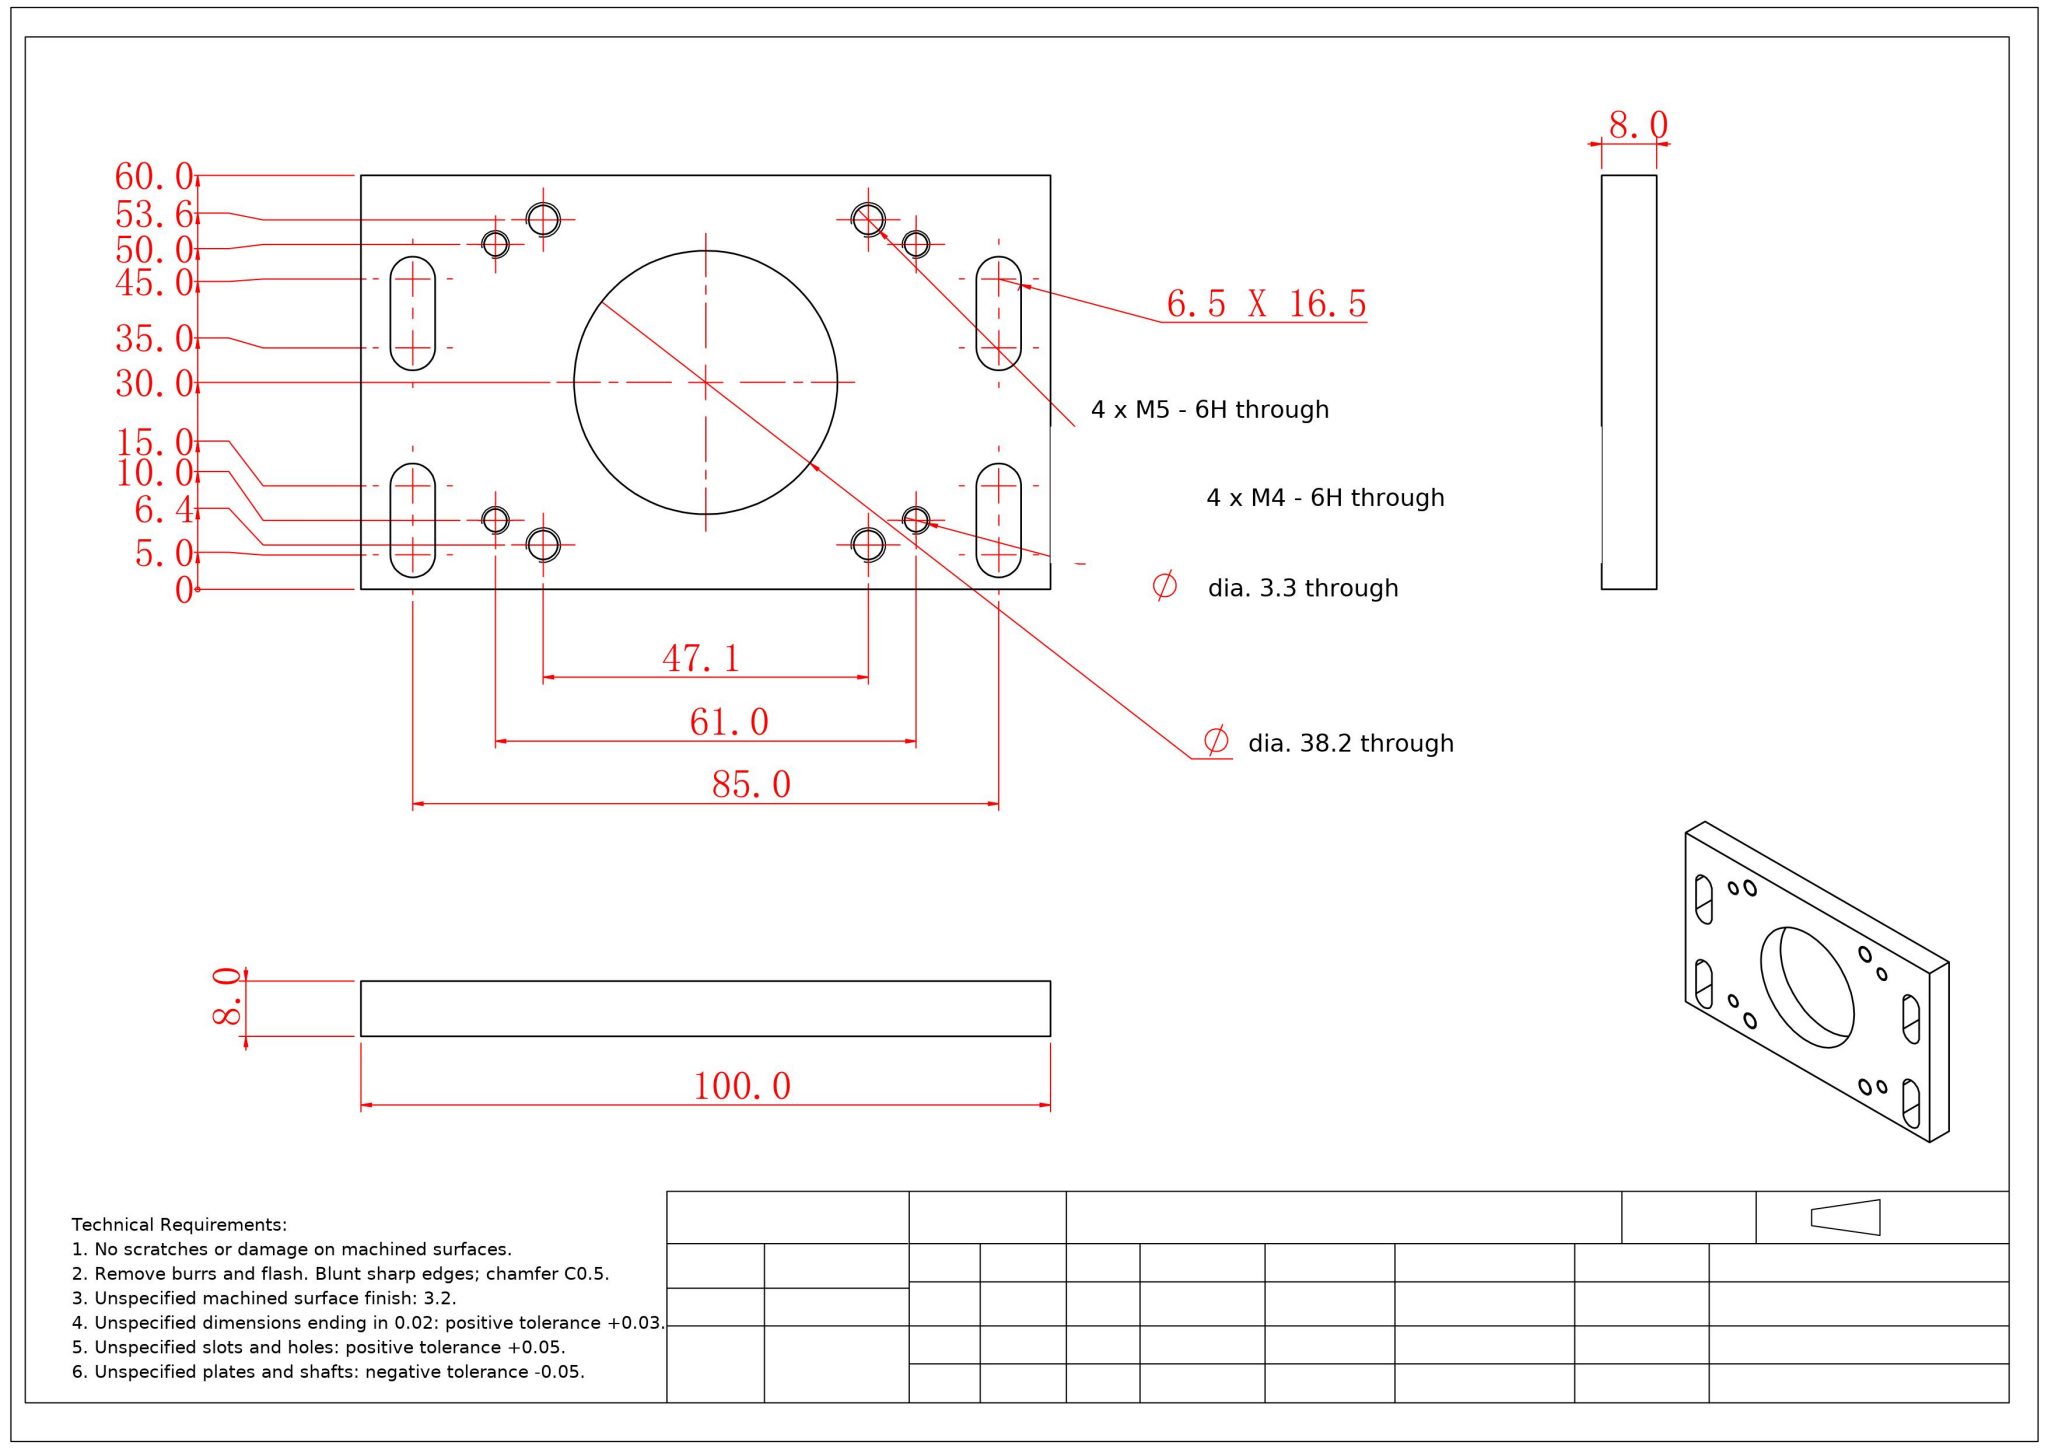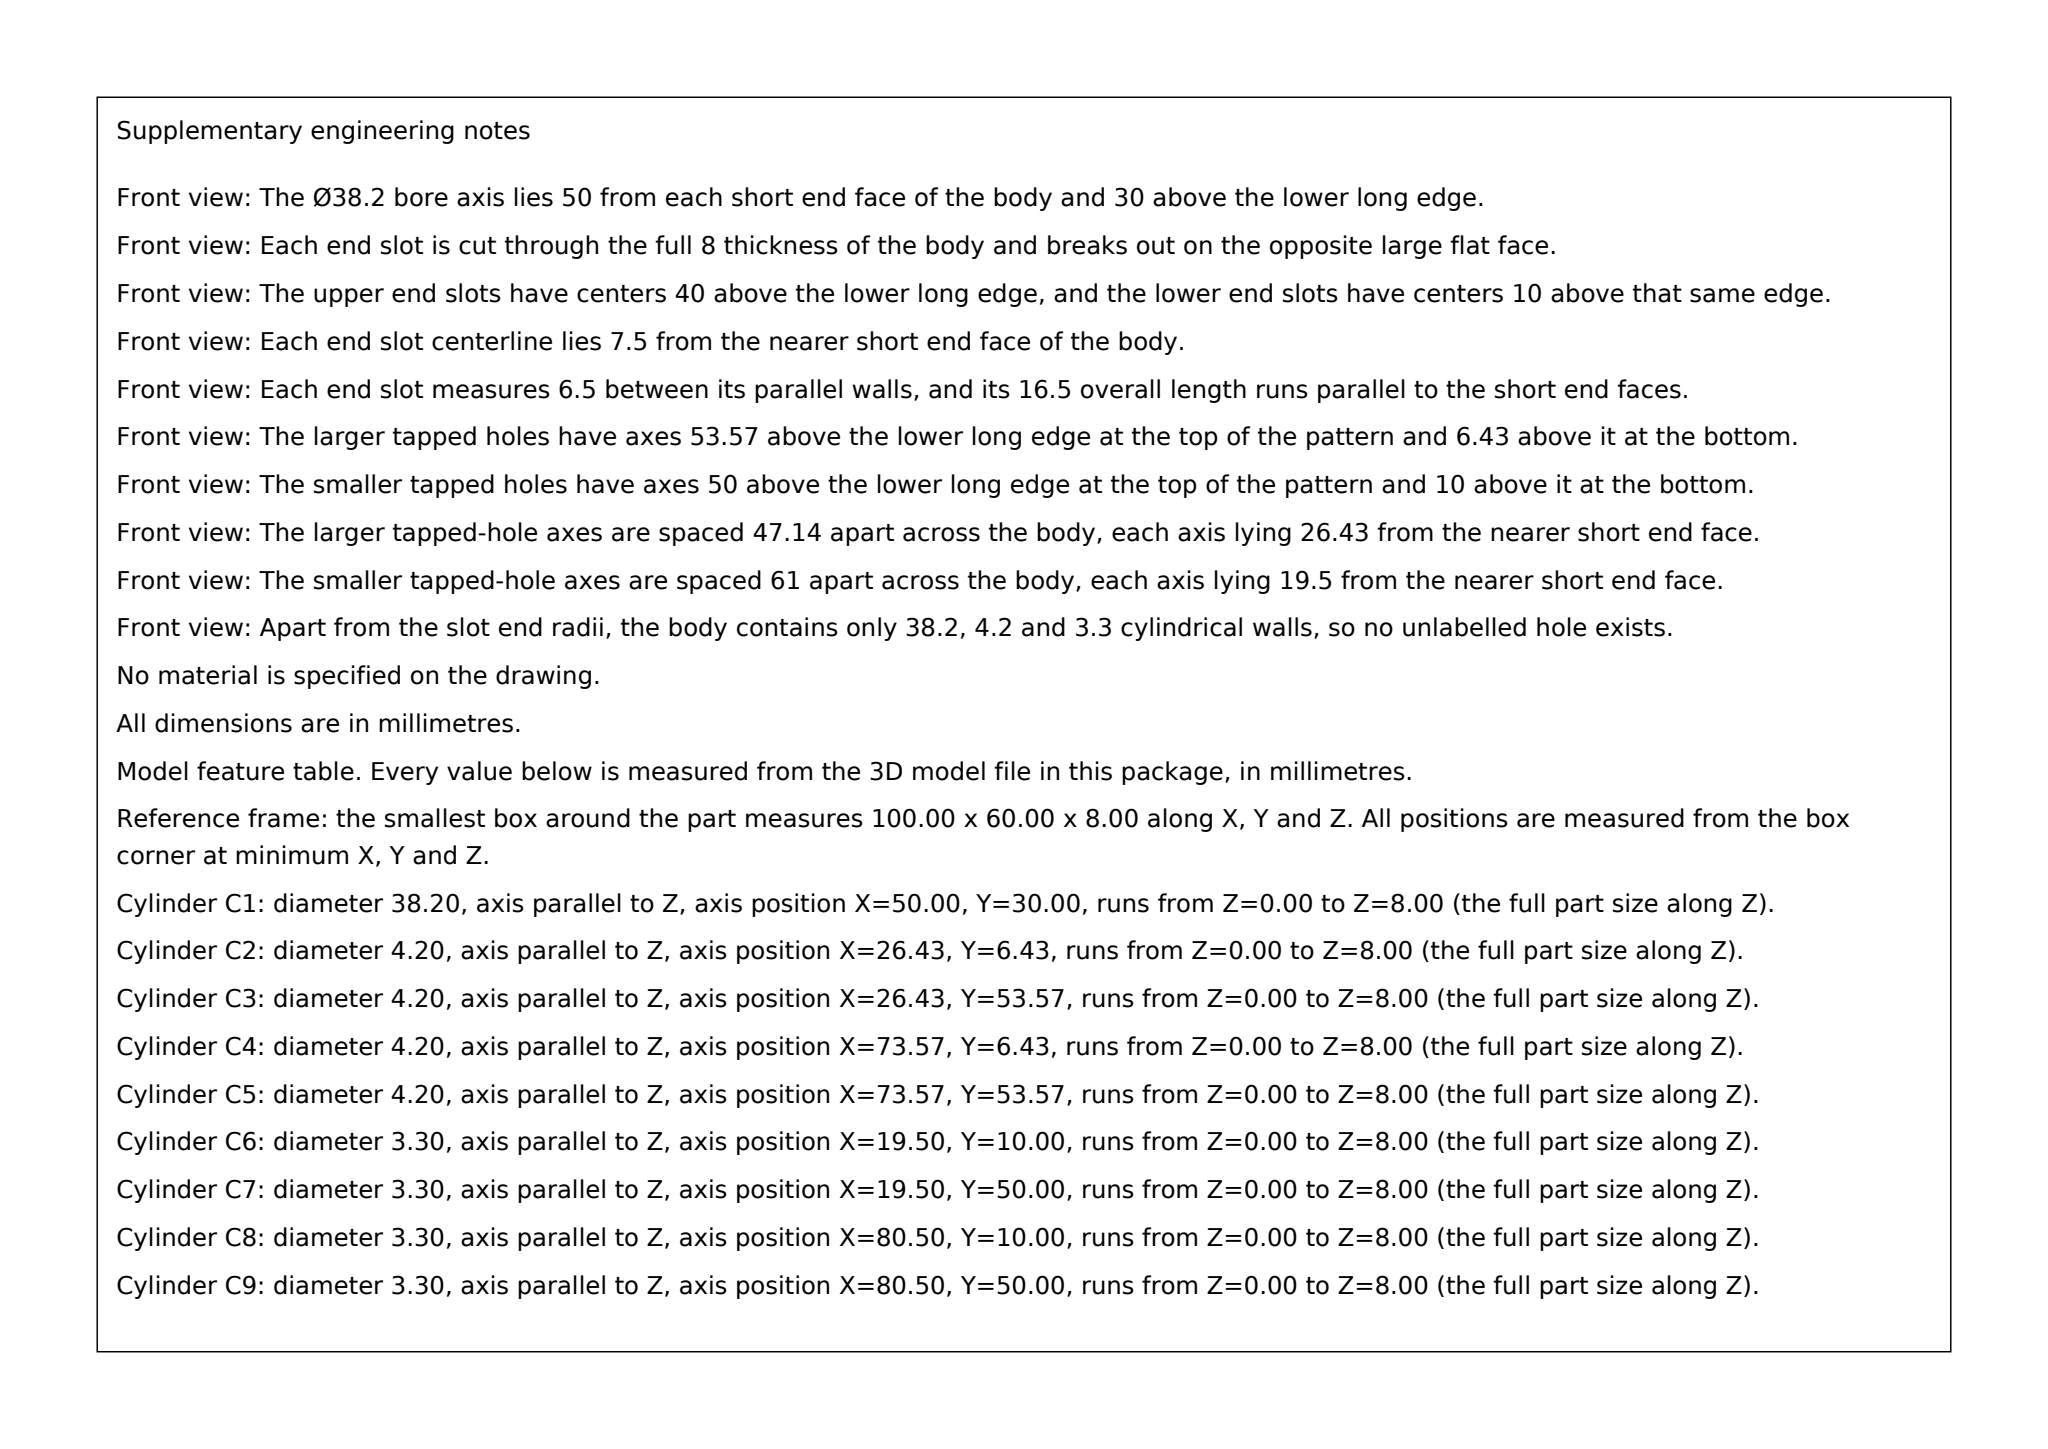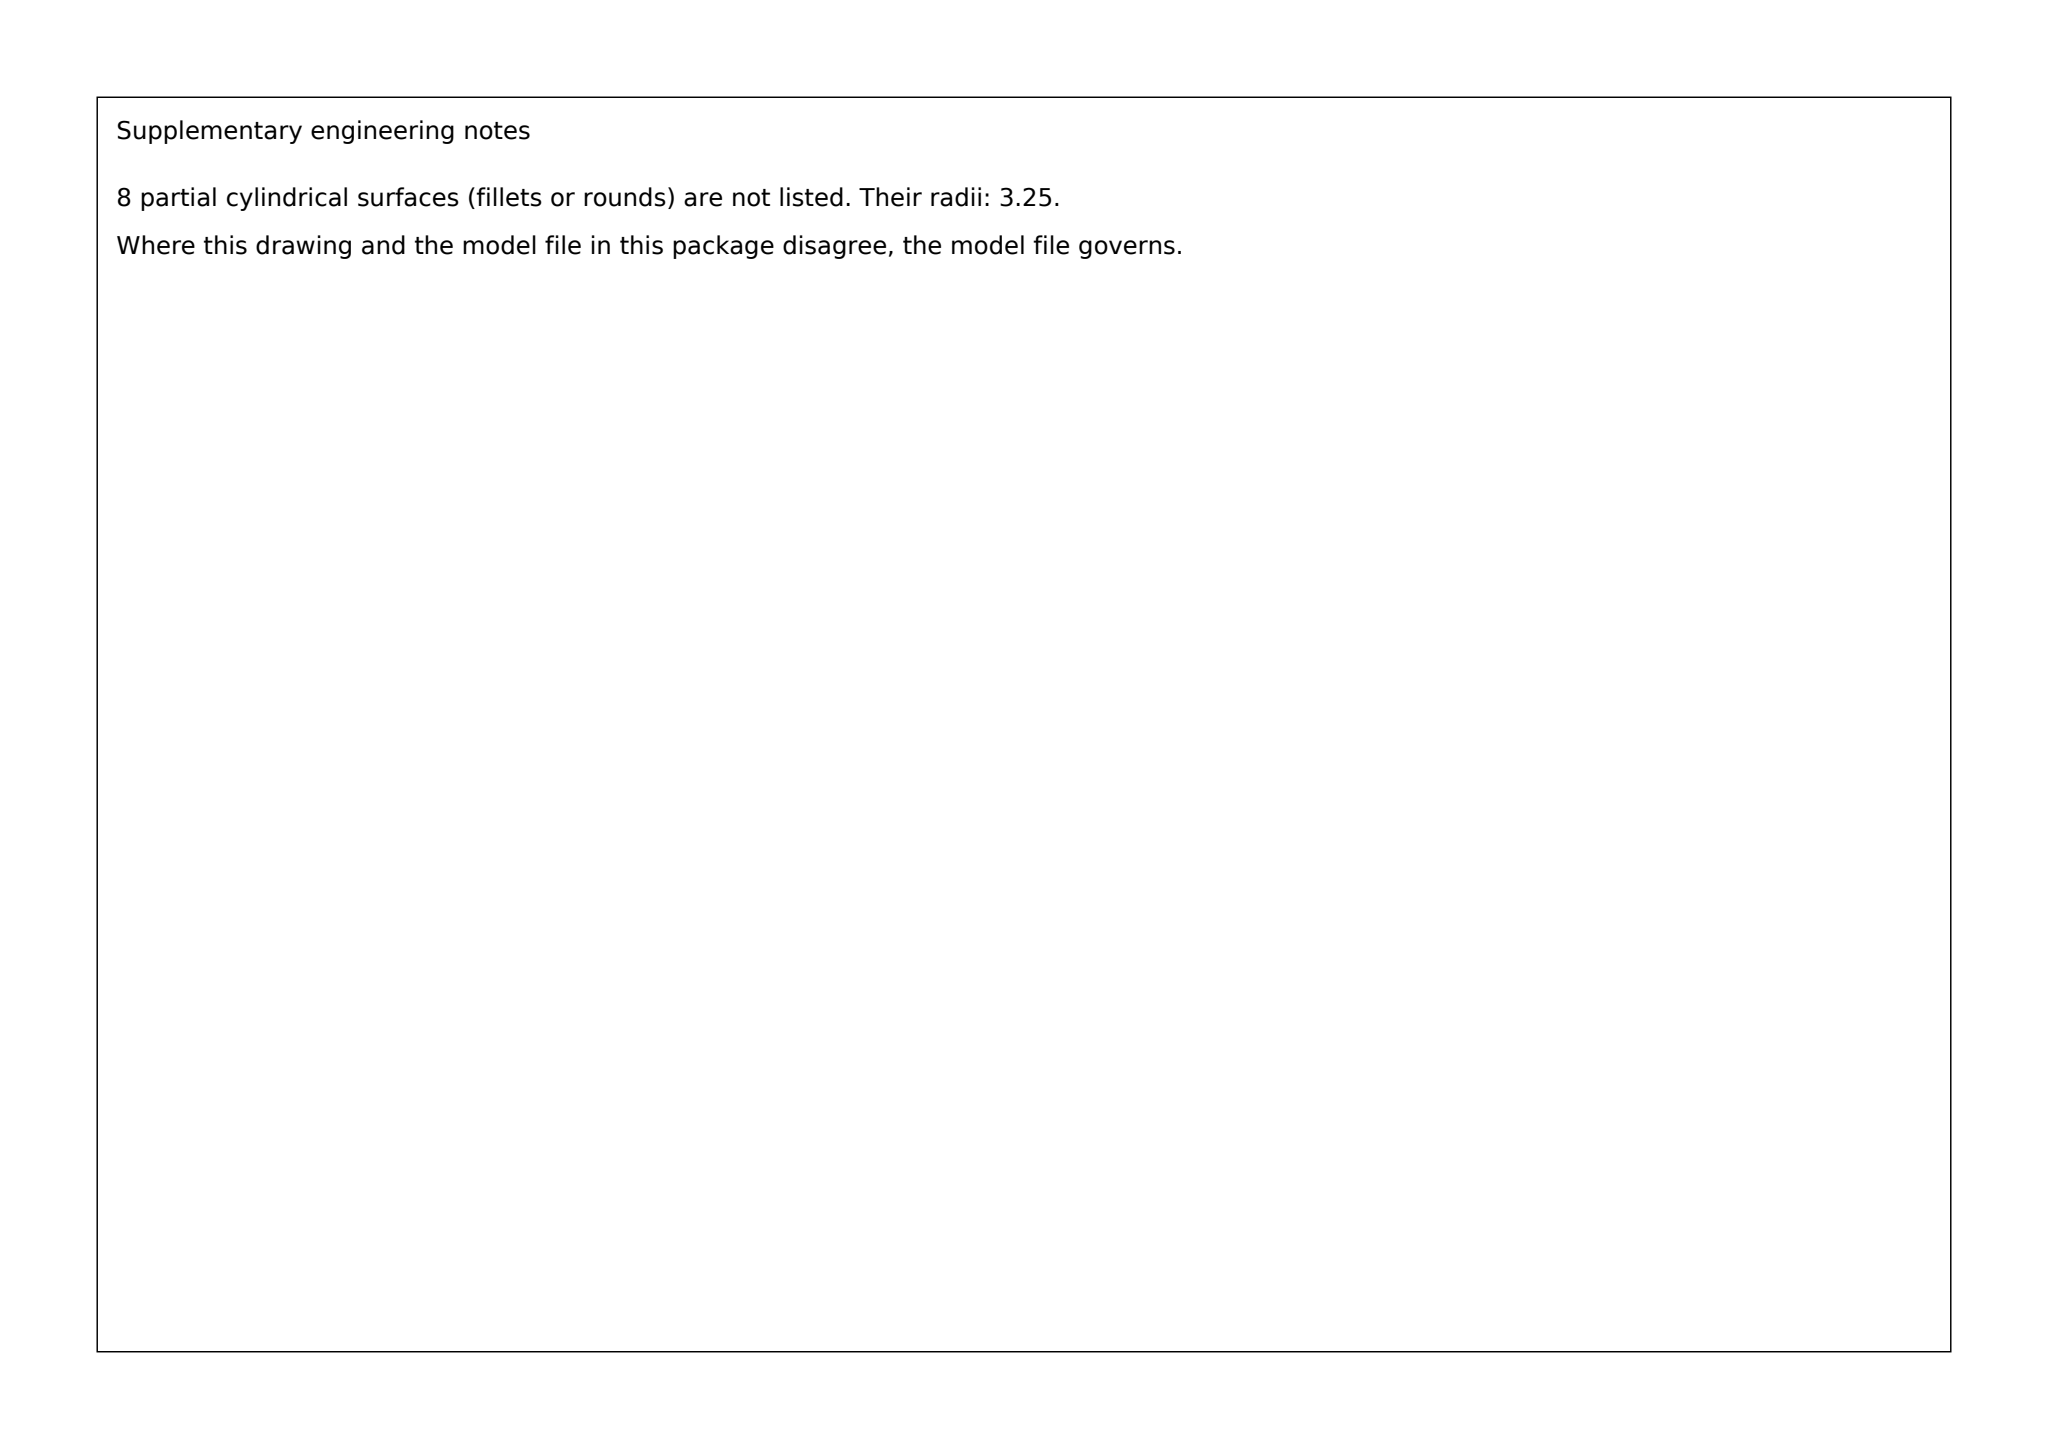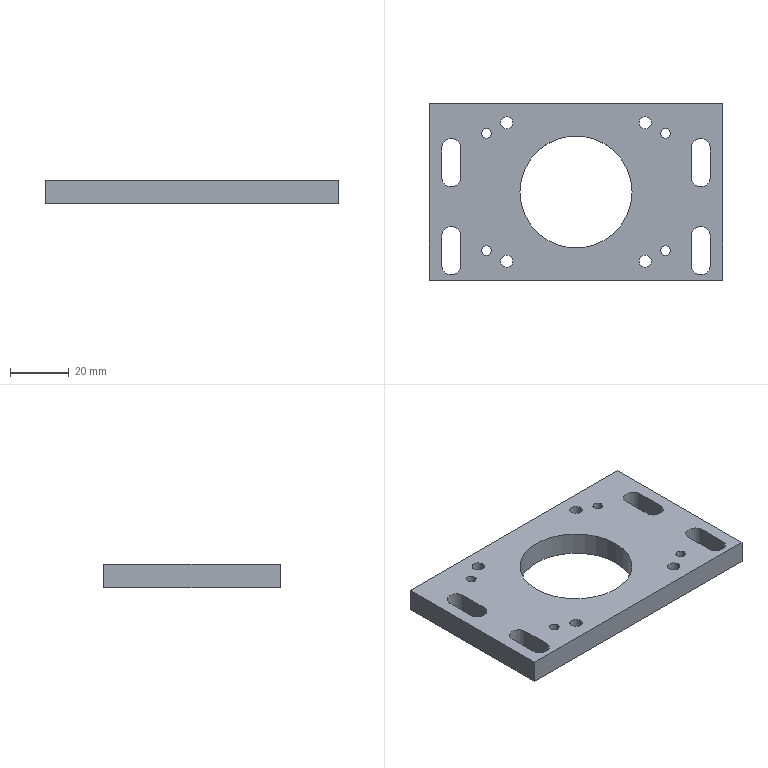Part | SolidWorks | mm | 1 solid | 40 faces | box 100 x 60 x 8 mm | volume 34972 mm3 | cylinder 26 | plane 14 | commonest cylinder face diameters 3.3 x8 4.2 x8 6.5 x8 38.2 x2
build123d program:
from build123d import *

# Parameters (mm, degrees)
SKETCH1_W           = 100
SKETCH1_H           = 60
BOSS_EXTRUDE1_DEPTH = 8
SKETCH2_R           = 19.1
CUT_EXTRUDE1_DEPTH  = 10
M5_TAPPED_HOLE1_D   = 4.2
CUT_EXTRUDE2_DEPTH  = 10
M4_TAPPED_HOLE1_D   = 3.3


with BuildPart() as part:
    # Sketch1 → Boss-Extrude1 (new body)
    with BuildSketch(Plane.XY):
        Rectangle(SKETCH1_W, SKETCH1_H)
    extrude(amount=BOSS_EXTRUDE1_DEPTH)

    # Sketch2 → Cut-Extrude1 (cut)
    with BuildSketch(Plane.XY.offset(8)):
        Circle(SKETCH2_R)
    extrude(amount=-CUT_EXTRUDE1_DEPTH, mode=Mode.SUBTRACT)

    # M5 Tapped Hole1 (through all)
    with Locations(Plane.XY.offset(8)):
        with Locations((-23.57, 23.57), (-23.57, -23.57), (23.57, -23.57), (23.57, 23.57)):
            Hole(M5_TAPPED_HOLE1_D / 2)

    # Sketch5 → Cut-Extrude2 (cut)
    with BuildSketch(Plane.XY.offset(8)):
        with BuildLine():
            Line((-39.25, 15), (-39.25, 5))
            ThreePointArc((-39.25, 5), (-42.5, 1.75), (-45.75, 5))
            Line((-45.75, 5), (-45.75, 15))
            ThreePointArc((-45.75, 15), (-42.5, 18.25), (-39.25, 15))
        make_face()
        with BuildLine():
            Line((-39.25, -15), (-39.25, -25))
            ThreePointArc((-39.25, -25), (-42.5, -28.25), (-45.75, -25))
            Line((-45.75, -25), (-45.75, -15))
            ThreePointArc((-45.75, -15), (-42.5, -11.75), (-39.25, -15))
        make_face()
        with BuildLine():
            Line((45.75, 15), (45.75, 5))
            ThreePointArc((45.75, 5), (42.5, 1.75), (39.25, 5))
            Line((39.25, 5), (39.25, 15))
            ThreePointArc((39.25, 15), (42.5, 18.25), (45.75, 15))
        make_face()
        with BuildLine():
            Line((45.75, -15), (45.75, -25))
            ThreePointArc((45.75, -25), (42.5, -28.25), (39.25, -25))
            Line((39.25, -25), (39.25, -15))
            ThreePointArc((39.25, -15), (42.5, -11.75), (45.75, -15))
        make_face()
    extrude(amount=-CUT_EXTRUDE2_DEPTH, mode=Mode.SUBTRACT)

    # M4 Tapped Hole1 (through all)
    with Locations(Plane.XY.offset(8)):
        with Locations((-30.5, -20), (-30.5, 20), (30.5, -20), (30.5, 20)):
            Hole(M4_TAPPED_HOLE1_D / 2)


solid = part.part